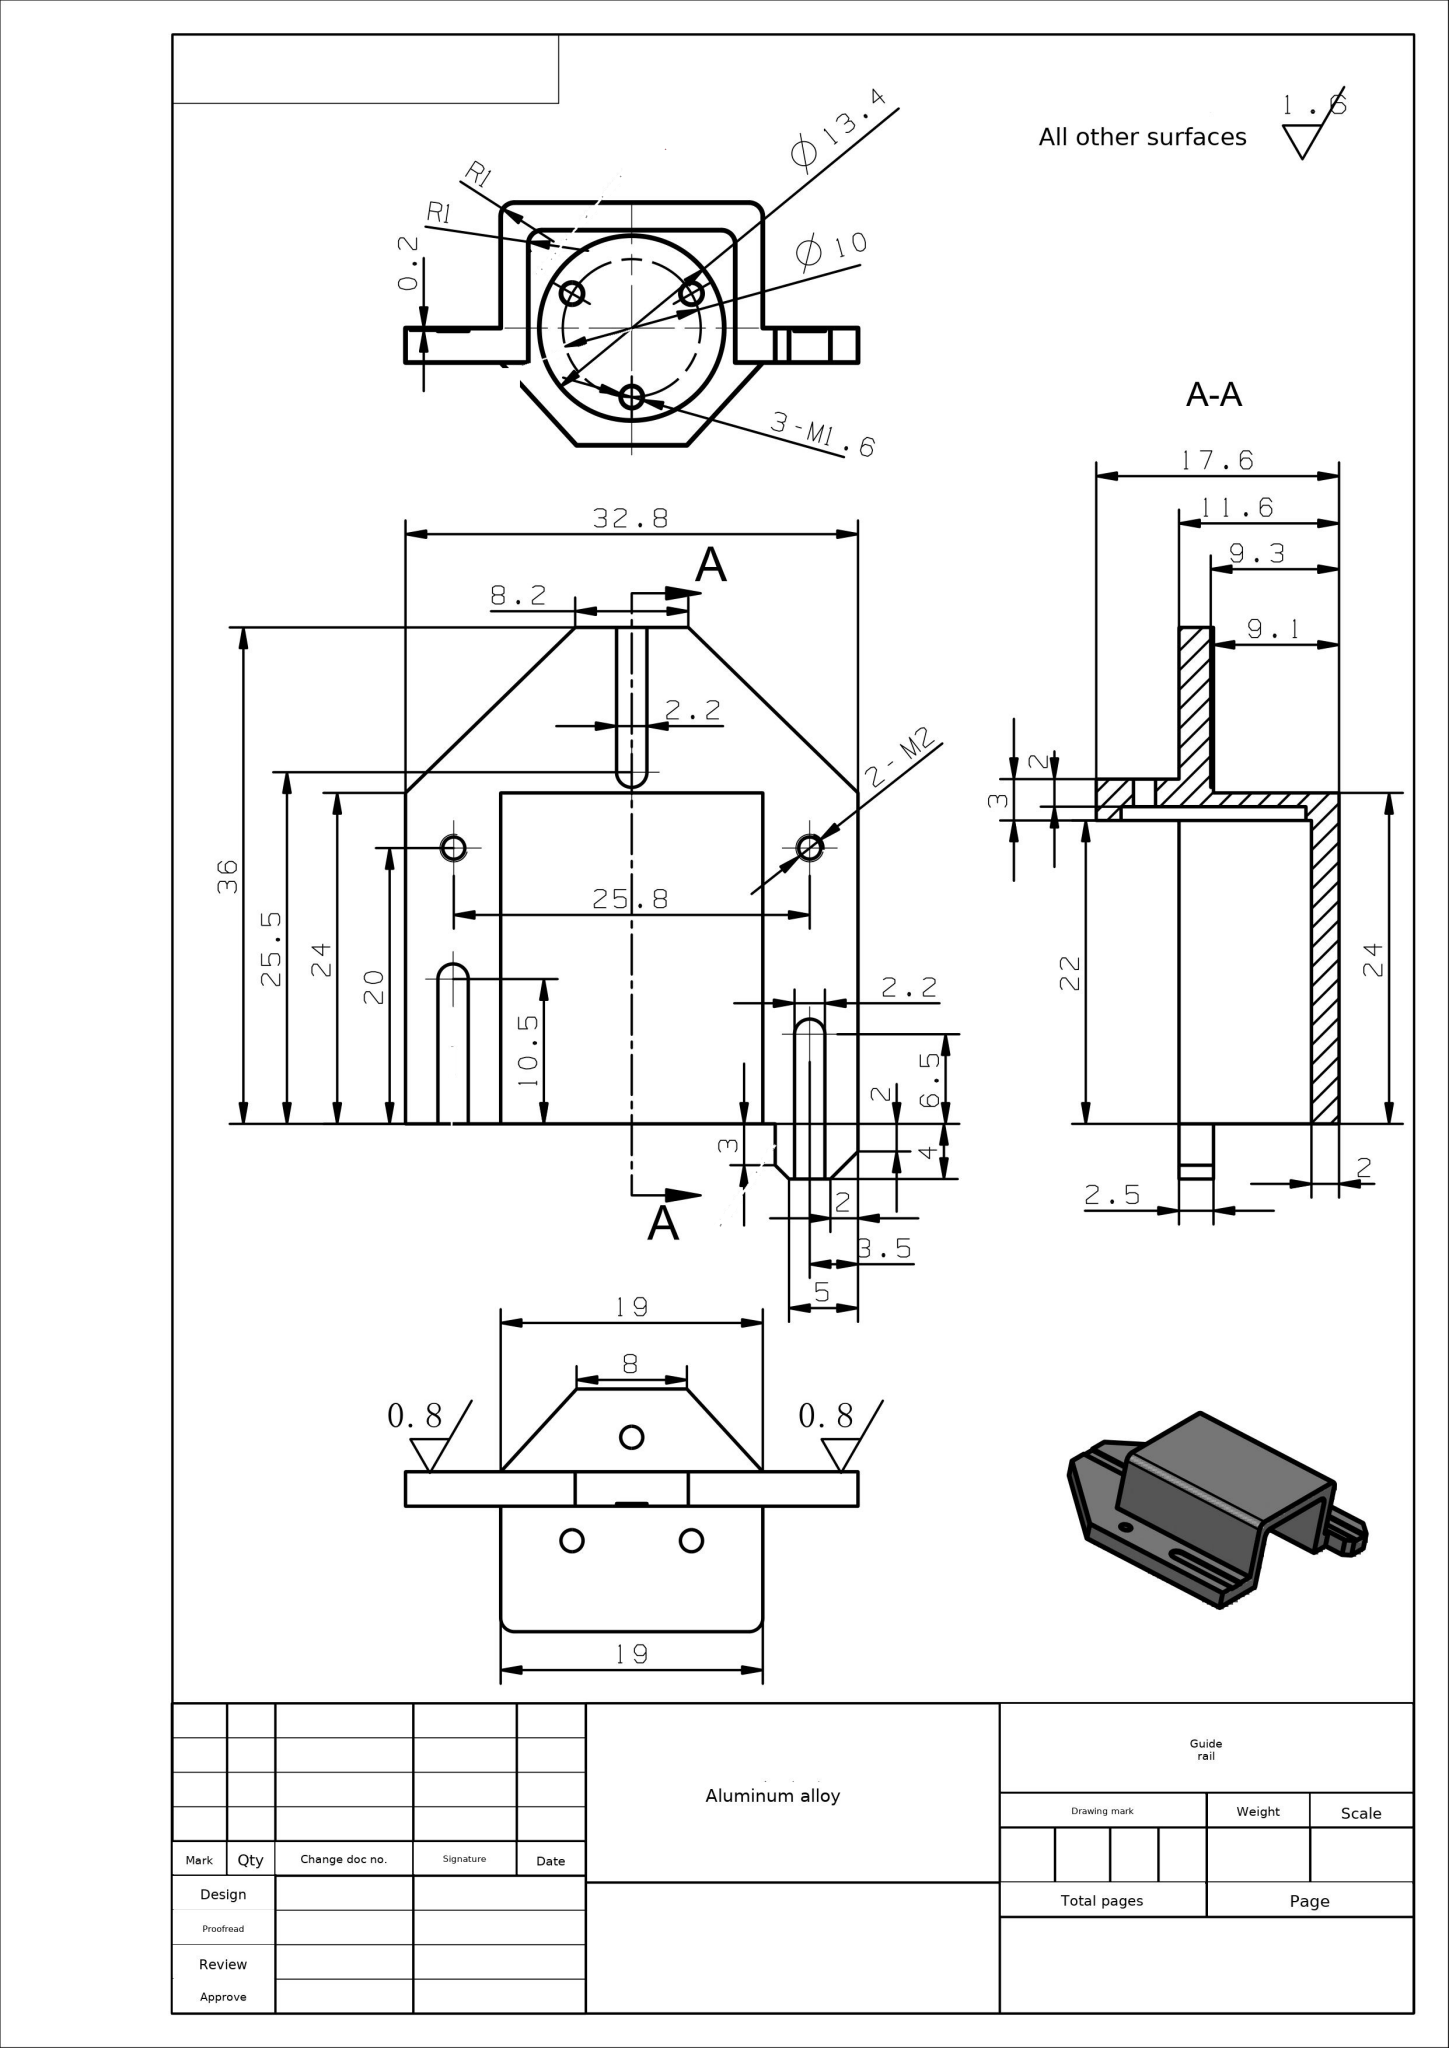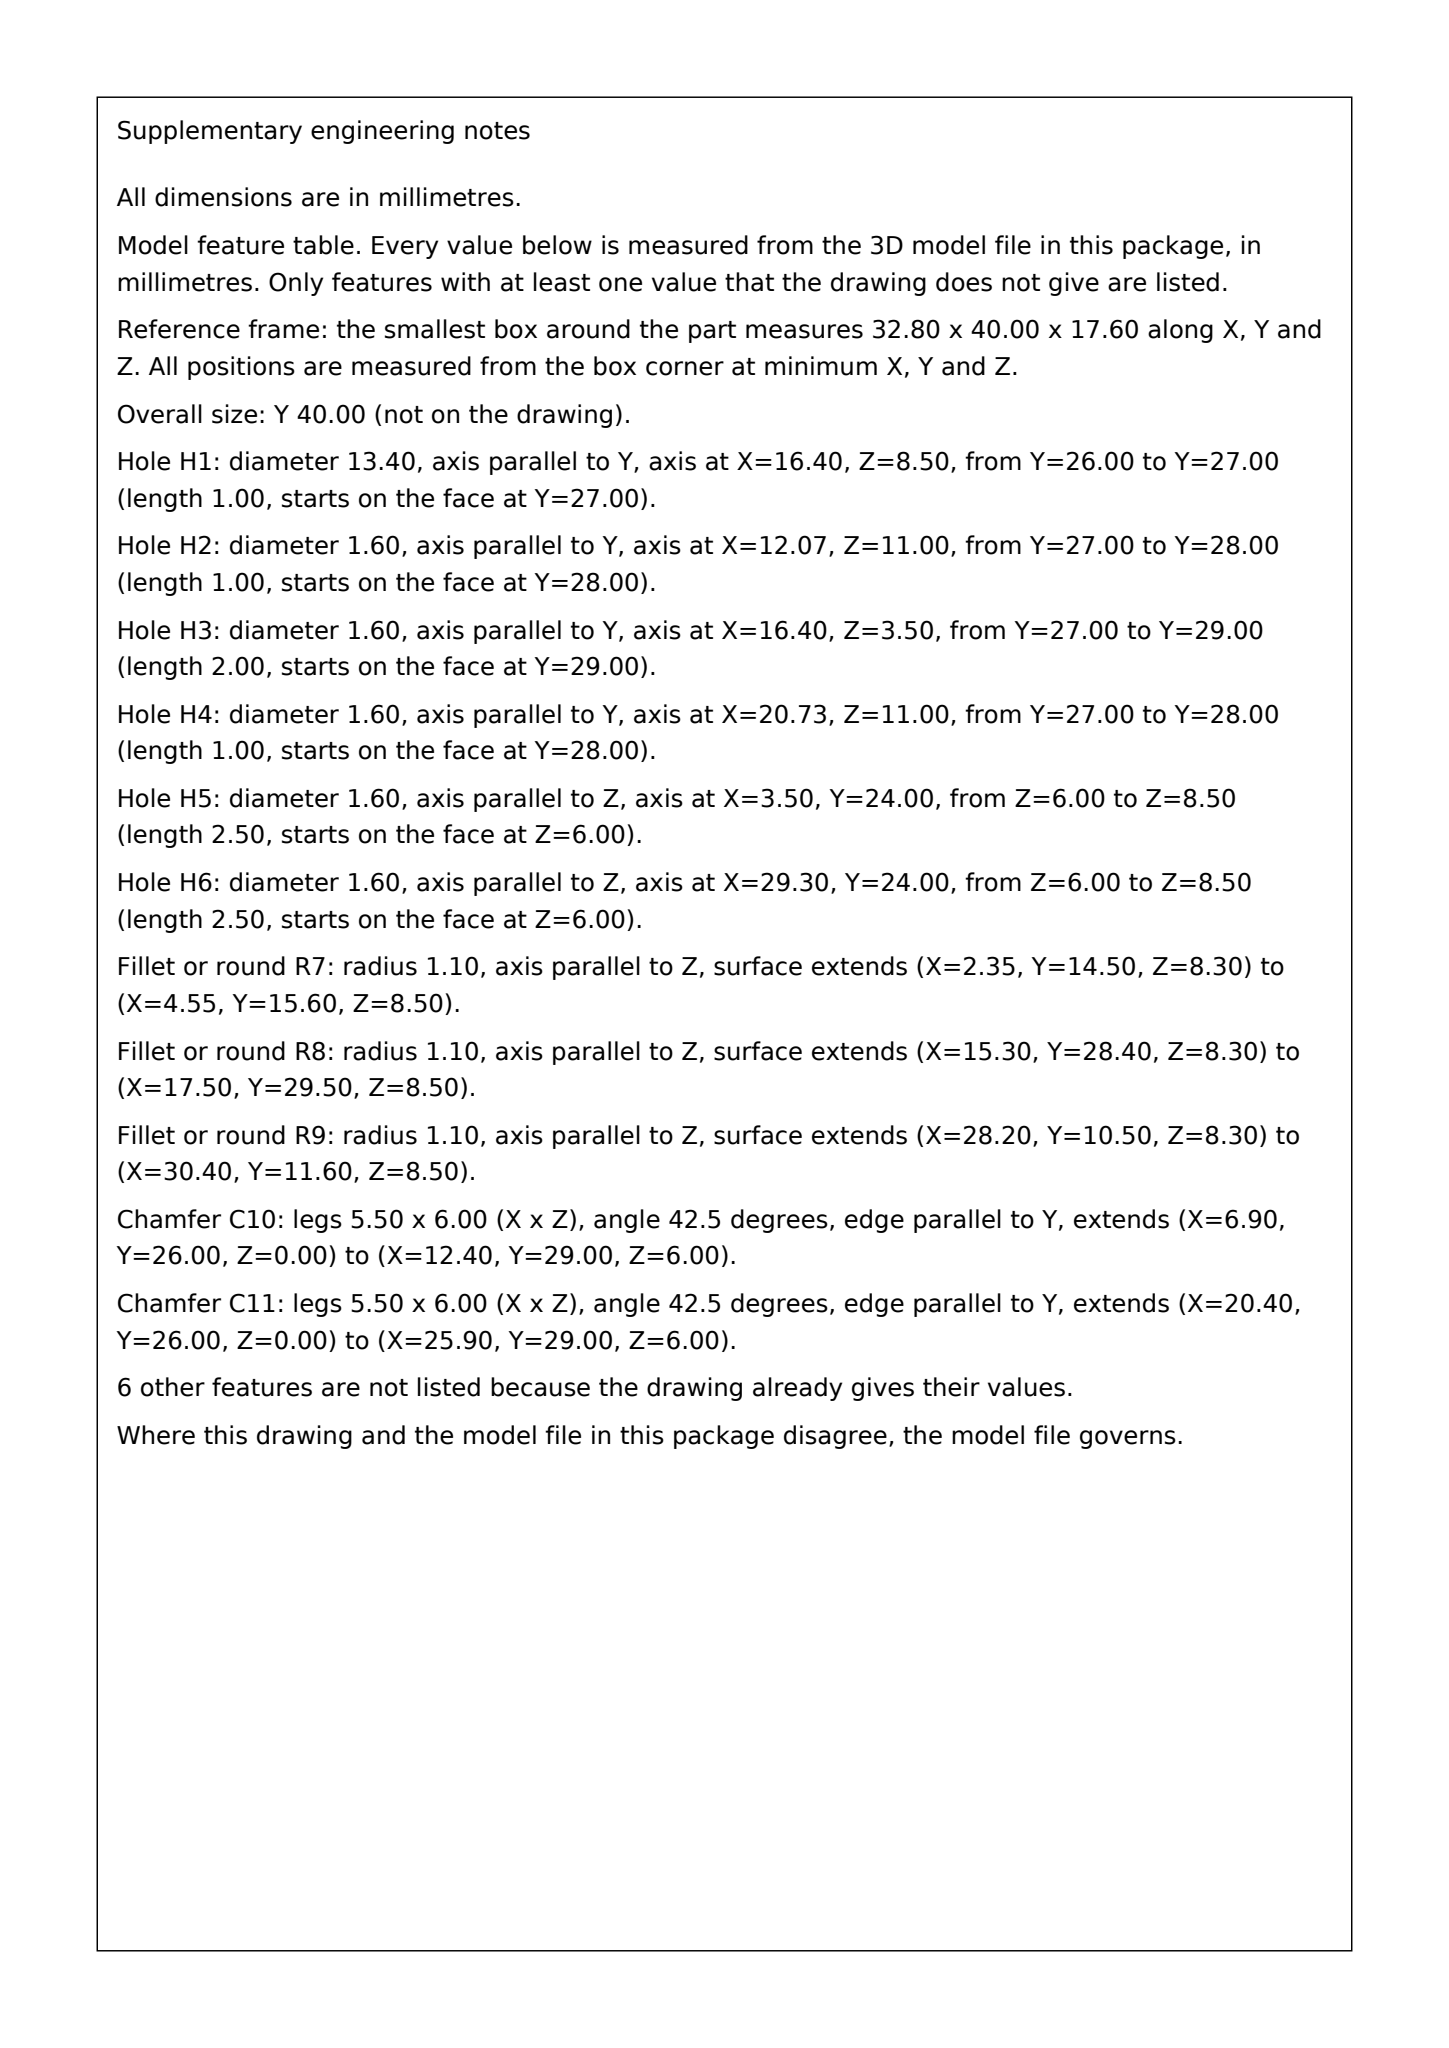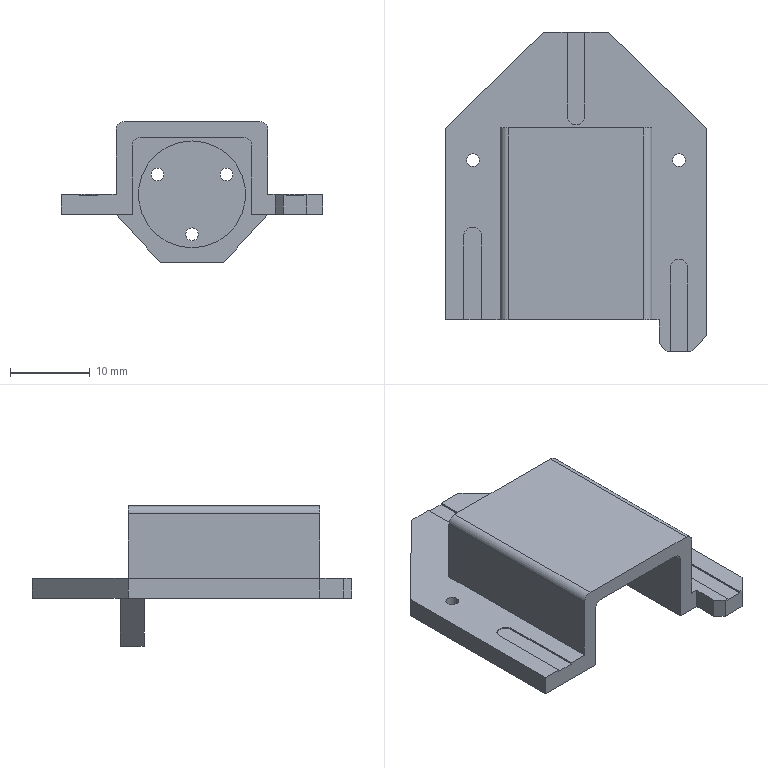Part | SolidWorks | mm | material Aluminum alloy | 1 solid | 53 faces | box 32.8 x 40 x 17.6 mm | volume 3686 mm3 | plane 34 | cylinder 19 | commonest cylinder face diameters 1.6 x10 2 x4 2.2 x3 13.4 x2